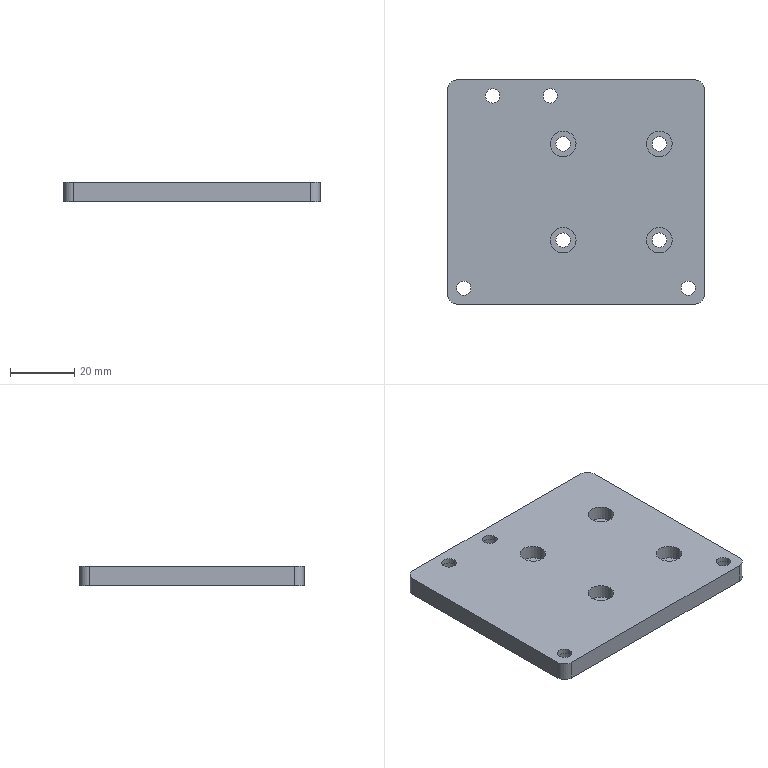CAM job | Mastercam | mm | 15 operations | part box 80 x 70 x 6
1. Facing | 24 - 80 平铣刀
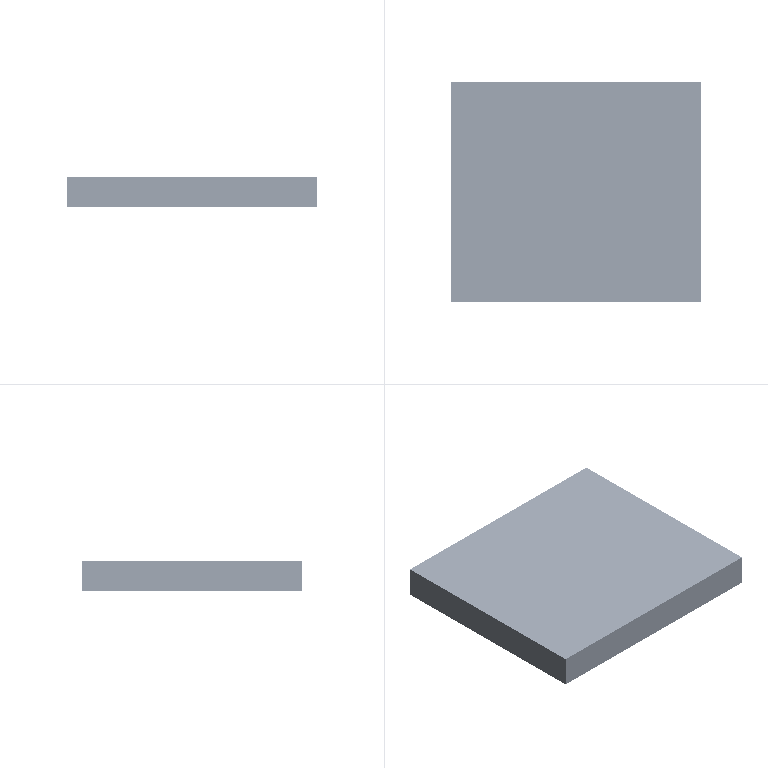2. 2D High Speed (2D Dynamic Mill) | 8 - 8C
3. Contour (2D) | 9 - 8J
4. Drill/Counterbore | 1 - 6 倒角刀
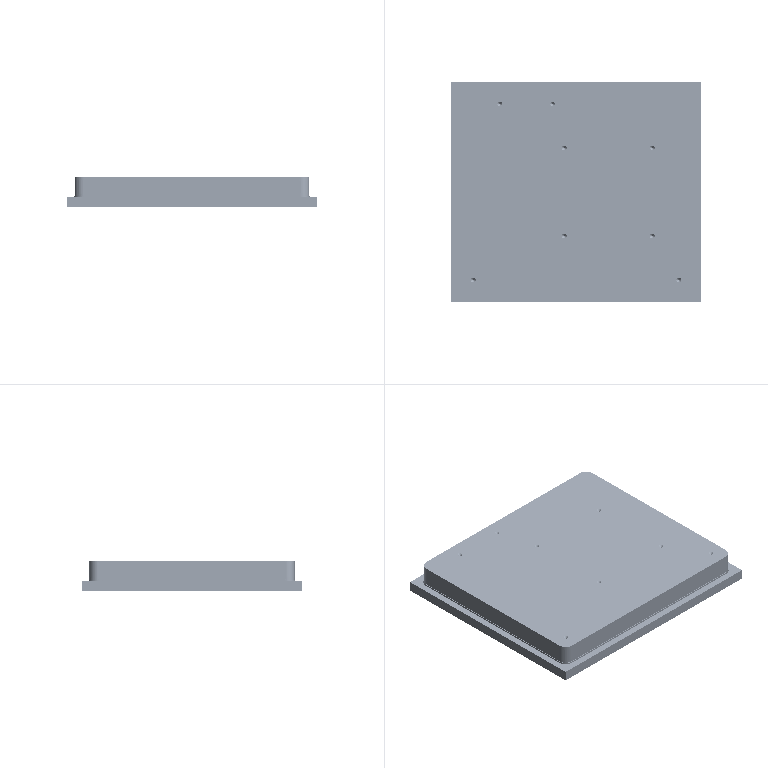5. Peck Drill | 32 - 4.5 钻头
6. Contour (Ramp) | 4 - 4C
7. Contour (2D) | 5 - 4J
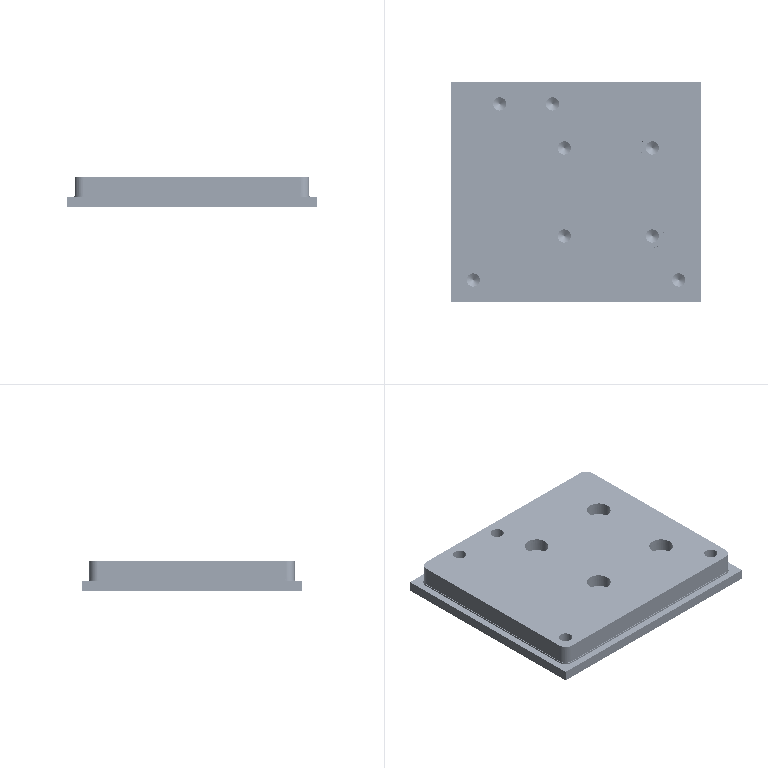8. Chamfer Drill | 1 - 6 倒角刀
9. Contour (2D chamfer) | 1 - 6 倒角刀
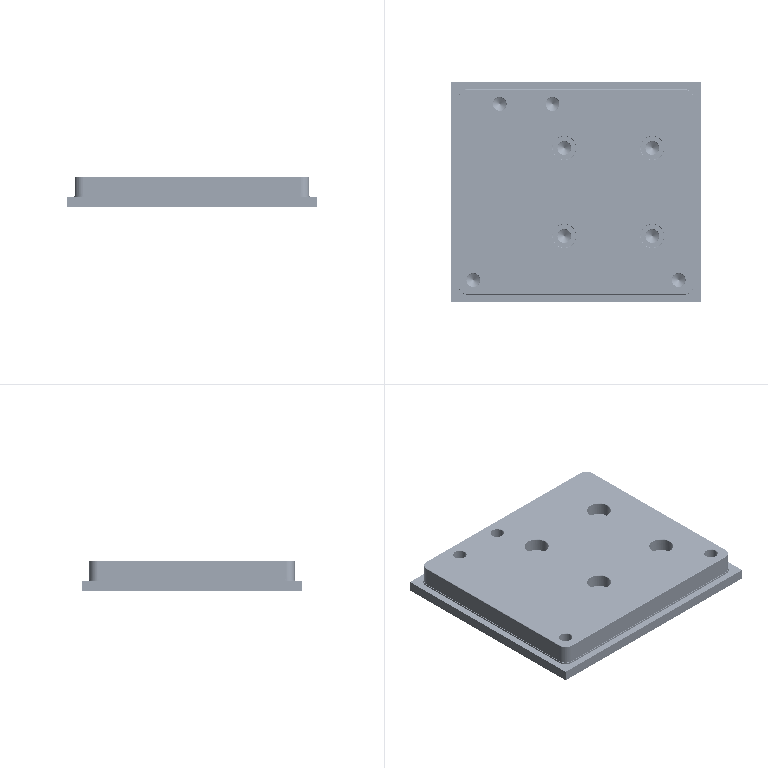10. Facing | 24 - 80 平铣刀
11. Facing | 24 - 80 平铣刀
12. Contour (Ramp) | 4 - 4C
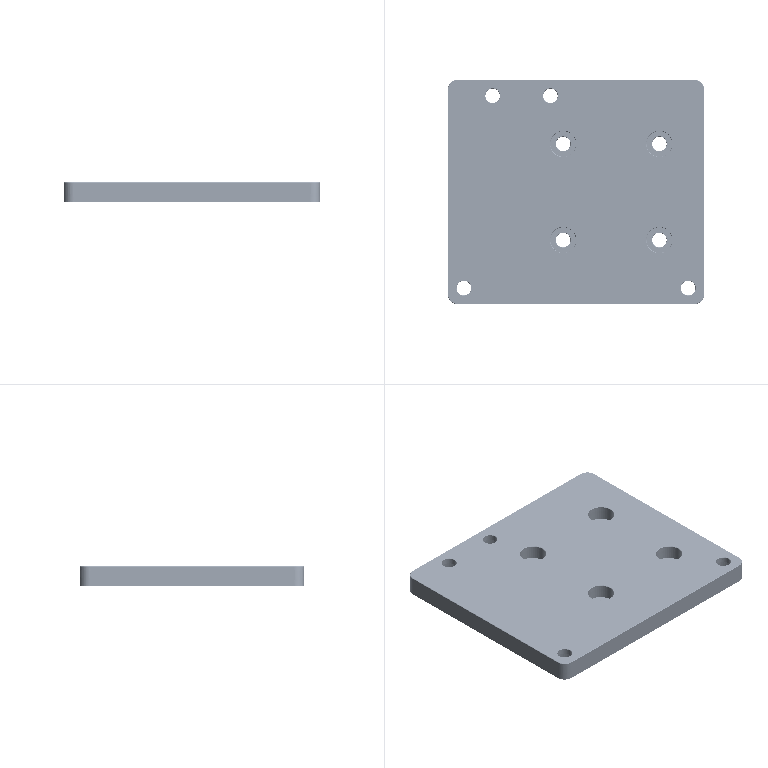13. Contour (2D) | 5 - 4J
14. Chamfer Drill | 1 - 6 倒角刀
15. Contour (2D chamfer) | 1 - 6 倒角刀